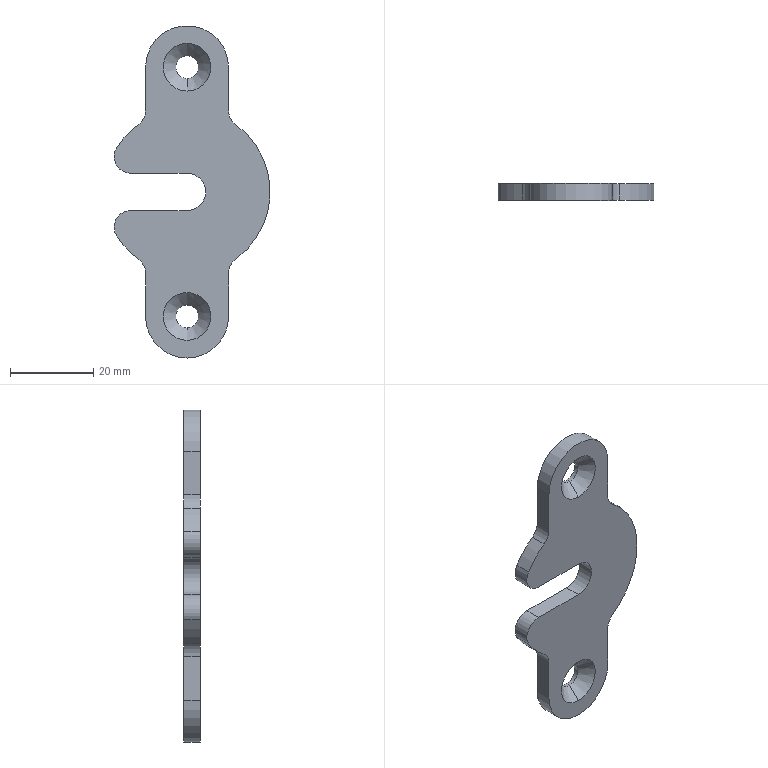Component | SolidWorks | QX1-16-BJPusherCylinderConnectionBlock-1 | 1 solid | 29 faces | box 37.56 x 4 x 80 mm | volume 6717 mm3 | cylinder 17 | plane 8 | cone 4 | commonest cylinder face diameters 8 x6 5.5 x4 20 x3 40 x3 9 x1 | material Q235
STEP:
#1=CARTESIAN_POINT('',(0.,-3.701,-1.289));
#2=VERTEX_POINT('',#1);
#3=CARTESIAN_POINT('',(0.,-3.701,-1.073));
#4=VERTEX_POINT('',#3);
#5=CARTESIAN_POINT('',(0.,-3.701,-1.181));
#6=DIRECTION('',(0.,-1.,0.));
#7=DIRECTION('',(0.,0.,-1.));
#8=AXIS2_PLACEMENT_3D('',#5,#6,#7);
#9=CIRCLE('',#8,0.1083);
#10=EDGE_CURVE('',#2,#4,#9,.T.);
#11=ORIENTED_EDGE('',*,*,#10,.F.);
#12=CARTESIAN_POINT('',(0.,-3.819,-1.407));
#13=VERTEX_POINT('',#12);
#14=CARTESIAN_POINT('',(0.,-3.701,-1.289));
#15=DIRECTION('',(0.,-0.7071,-0.7071));
#16=VECTOR('',#15,39.37);
#17=LINE('',#14,#16);
#18=EDGE_CURVE('',#2,#13,#17,.T.);
#19=ORIENTED_EDGE('',*,*,#18,.T.);
#20=CARTESIAN_POINT('',(0.,-3.819,-0.9547));
#21=VERTEX_POINT('',#20);
#22=CARTESIAN_POINT('',(0.,-3.819,-1.181));
#23=DIRECTION('',(-0.,1.,-0.));
#24=DIRECTION('',(0.,0.,-1.));
#25=AXIS2_PLACEMENT_3D('',#22,#23,#24);
#26=CIRCLE('',#25,0.2264);
#27=EDGE_CURVE('',#21,#13,#26,.T.);
#28=ORIENTED_EDGE('',*,*,#27,.F.);
#29=CARTESIAN_POINT('',(0.,-3.701,-1.073));
#30=DIRECTION('',(0.,-0.7071,0.7071));
#31=VECTOR('',#30,39.37);
#32=LINE('',#29,#31);
#33=EDGE_CURVE('',#4,#21,#32,.T.);
#34=ORIENTED_EDGE('',*,*,#33,.F.);
#35=EDGE_LOOP('',(#11,#19,#28,#34));
#36=FACE_OUTER_BOUND('',#35,.T.);
#37=CARTESIAN_POINT('',(0.,-3.701,-1.181));
#38=DIRECTION('',(0.,-1.,0.));
#39=DIRECTION('',(-0.,0.,1.));
#40=AXIS2_PLACEMENT_3D('',#37,#38,#39);
#41=CONICAL_SURFACE('',#40,0.1083,0.7854);
#42=ADVANCED_FACE('',(#36),#41,.F.);
#43=CARTESIAN_POINT('',(0.,-3.701,1.073));
#44=VERTEX_POINT('',#43);
#45=CARTESIAN_POINT('',(0.,-3.701,1.289));
#46=VERTEX_POINT('',#45);
#47=CARTESIAN_POINT('',(0.,-3.701,1.181));
#48=DIRECTION('',(0.,-1.,0.));
#49=DIRECTION('',(0.,0.,-1.));
#50=AXIS2_PLACEMENT_3D('',#47,#48,#49);
#51=CIRCLE('',#50,0.1083);
#52=EDGE_CURVE('',#44,#46,#51,.T.);
#53=ORIENTED_EDGE('',*,*,#52,.F.);
#54=CARTESIAN_POINT('',(0.,-3.819,0.9547));
#55=VERTEX_POINT('',#54);
#56=CARTESIAN_POINT('',(0.,-3.701,1.073));
#57=DIRECTION('',(0.,-0.7071,-0.7071));
#58=VECTOR('',#57,39.37);
#59=LINE('',#56,#58);
#60=EDGE_CURVE('',#44,#55,#59,.T.);
#61=ORIENTED_EDGE('',*,*,#60,.T.);
#62=CARTESIAN_POINT('',(0.,-3.819,1.407));
#63=VERTEX_POINT('',#62);
#64=CARTESIAN_POINT('',(0.,-3.819,1.181));
#65=DIRECTION('',(-0.,1.,-0.));
#66=DIRECTION('',(0.,0.,-1.));
#67=AXIS2_PLACEMENT_3D('',#64,#65,#66);
#68=CIRCLE('',#67,0.2264);
#69=EDGE_CURVE('',#63,#55,#68,.T.);
#70=ORIENTED_EDGE('',*,*,#69,.F.);
#71=CARTESIAN_POINT('',(0.,-3.701,1.289));
#72=DIRECTION('',(0.,-0.7071,0.7071));
#73=VECTOR('',#72,39.37);
#74=LINE('',#71,#73);
#75=EDGE_CURVE('',#46,#63,#74,.T.);
#76=ORIENTED_EDGE('',*,*,#75,.F.);
#77=EDGE_LOOP('',(#53,#61,#70,#76));
#78=FACE_OUTER_BOUND('',#77,.T.);
#79=CARTESIAN_POINT('',(0.,-3.701,1.181));
#80=DIRECTION('',(0.,-1.,0.));
#81=DIRECTION('',(-0.,0.,1.));
#82=AXIS2_PLACEMENT_3D('',#79,#80,#81);
#83=CONICAL_SURFACE('',#82,0.1083,0.7854);
#84=ADVANCED_FACE('',(#78),#83,.F.);
#85=CARTESIAN_POINT('',(0.,-3.661,-1.289));
#86=VERTEX_POINT('',#85);
#87=CARTESIAN_POINT('',(0.,-3.661,-1.073));
#88=VERTEX_POINT('',#87);
#89=CARTESIAN_POINT('',(0.,-3.661,-1.181));
#90=DIRECTION('',(0.,-1.,0.));
#91=DIRECTION('',(-0.,0.,1.));
#92=AXIS2_PLACEMENT_3D('',#89,#90,#91);
#93=CIRCLE('',#92,0.1083);
#94=EDGE_CURVE('',#86,#88,#93,.T.);
#95=ORIENTED_EDGE('',*,*,#94,.F.);
#96=CARTESIAN_POINT('',(0.,-3.819,-1.289));
#97=DIRECTION('',(0.,-1.,0.));
#98=VECTOR('',#97,39.37);
#99=LINE('',#96,#98);
#100=EDGE_CURVE('',#86,#2,#99,.T.);
#101=ORIENTED_EDGE('',*,*,#100,.T.);
#102=ORIENTED_EDGE('',*,*,#10,.T.);
#103=CARTESIAN_POINT('',(0.,-3.819,-1.073));
#104=DIRECTION('',(0.,-1.,0.));
#105=VECTOR('',#104,39.37);
#106=LINE('',#103,#105);
#107=EDGE_CURVE('',#88,#4,#106,.T.);
#108=ORIENTED_EDGE('',*,*,#107,.F.);
#109=EDGE_LOOP('',(#95,#101,#102,#108));
#110=FACE_OUTER_BOUND('',#109,.T.);
#111=CARTESIAN_POINT('',(0.,-3.819,-1.181));
#112=DIRECTION('',(0.,-1.,0.));
#113=DIRECTION('',(-0.,0.,1.));
#114=AXIS2_PLACEMENT_3D('',#111,#112,#113);
#115=CYLINDRICAL_SURFACE('',#114,0.1083);
#116=ADVANCED_FACE('',(#110),#115,.F.);
#117=CARTESIAN_POINT('',(0.,-3.661,1.073));
#118=VERTEX_POINT('',#117);
#119=CARTESIAN_POINT('',(0.,-3.661,1.289));
#120=VERTEX_POINT('',#119);
#121=CARTESIAN_POINT('',(0.,-3.661,1.181));
#122=DIRECTION('',(0.,-1.,0.));
#123=DIRECTION('',(-0.,0.,1.));
#124=AXIS2_PLACEMENT_3D('',#121,#122,#123);
#125=CIRCLE('',#124,0.1083);
#126=EDGE_CURVE('',#118,#120,#125,.T.);
#127=ORIENTED_EDGE('',*,*,#126,.F.);
#128=CARTESIAN_POINT('',(0.,-3.819,1.073));
#129=DIRECTION('',(0.,-1.,0.));
#130=VECTOR('',#129,39.37);
#131=LINE('',#128,#130);
#132=EDGE_CURVE('',#118,#44,#131,.T.);
#133=ORIENTED_EDGE('',*,*,#132,.T.);
#134=ORIENTED_EDGE('',*,*,#52,.T.);
#135=CARTESIAN_POINT('',(0.,-3.819,1.289));
#136=DIRECTION('',(0.,-1.,0.));
#137=VECTOR('',#136,39.37);
#138=LINE('',#135,#137);
#139=EDGE_CURVE('',#120,#46,#138,.T.);
#140=ORIENTED_EDGE('',*,*,#139,.F.);
#141=EDGE_LOOP('',(#127,#133,#134,#140));
#142=FACE_OUTER_BOUND('',#141,.T.);
#143=CARTESIAN_POINT('',(0.,-3.819,1.181));
#144=DIRECTION('',(0.,-1.,0.));
#145=DIRECTION('',(-0.,0.,1.));
#146=AXIS2_PLACEMENT_3D('',#143,#144,#145);
#147=CYLINDRICAL_SURFACE('',#146,0.1083);
#148=ADVANCED_FACE('',(#142),#147,.F.);
#149=CARTESIAN_POINT('',(0.3937,-3.819,-1.181));
#150=VERTEX_POINT('',#149);
#151=CARTESIAN_POINT('',(0.,-3.819,-1.575));
#152=VERTEX_POINT('',#151);
#153=CARTESIAN_POINT('',(0.,-3.819,-1.181));
#154=DIRECTION('',(-0.,1.,-0.));
#155=DIRECTION('',(0.,0.,-1.));
#156=AXIS2_PLACEMENT_3D('',#153,#154,#155);
#157=CIRCLE('',#156,0.3937);
#158=EDGE_CURVE('',#150,#152,#157,.T.);
#159=ORIENTED_EDGE('',*,*,#158,.T.);
#160=CARTESIAN_POINT('',(0.,-3.661,-1.575));
#161=VERTEX_POINT('',#160);
#162=CARTESIAN_POINT('',(0.,-3.819,-1.575));
#163=DIRECTION('',(-0.,1.,-0.));
#164=VECTOR('',#163,39.37);
#165=LINE('',#162,#164);
#166=EDGE_CURVE('',#152,#161,#165,.T.);
#167=ORIENTED_EDGE('',*,*,#166,.T.);
#168=CARTESIAN_POINT('',(0.3937,-3.661,-1.181));
#169=VERTEX_POINT('',#168);
#170=CARTESIAN_POINT('',(0.,-3.661,-1.181));
#171=DIRECTION('',(-0.,1.,-0.));
#172=DIRECTION('',(0.,0.,-1.));
#173=AXIS2_PLACEMENT_3D('',#170,#171,#172);
#174=CIRCLE('',#173,0.3937);
#175=EDGE_CURVE('',#169,#161,#174,.T.);
#176=ORIENTED_EDGE('',*,*,#175,.F.);
#177=CARTESIAN_POINT('',(0.3937,-3.819,-1.181));
#178=DIRECTION('',(-0.,1.,-0.));
#179=VECTOR('',#178,39.37);
#180=LINE('',#177,#179);
#181=EDGE_CURVE('',#150,#169,#180,.T.);
#182=ORIENTED_EDGE('',*,*,#181,.F.);
#183=EDGE_LOOP('',(#159,#167,#176,#182));
#184=FACE_OUTER_BOUND('',#183,.T.);
#185=CARTESIAN_POINT('',(0.,-3.819,-1.181));
#186=DIRECTION('',(-0.,1.,-0.));
#187=DIRECTION('',(0.,0.,-1.));
#188=AXIS2_PLACEMENT_3D('',#185,#186,#187);
#189=CYLINDRICAL_SURFACE('',#188,0.3937);
#190=ADVANCED_FACE('',(#184),#189,.T.);
#191=ORIENTED_EDGE('',*,*,#69,.T.);
#192=CARTESIAN_POINT('',(0.,-3.819,1.181));
#193=DIRECTION('',(-0.,1.,-0.));
#194=DIRECTION('',(0.,0.,-1.));
#195=AXIS2_PLACEMENT_3D('',#192,#193,#194);
#196=CIRCLE('',#195,0.2264);
#197=EDGE_CURVE('',#55,#63,#196,.T.);
#198=ORIENTED_EDGE('',*,*,#197,.T.);
#199=EDGE_LOOP('',(#191,#198));
#200=FACE_BOUND('',#199,.T.);
#201=ORIENTED_EDGE('',*,*,#27,.T.);
#202=CARTESIAN_POINT('',(0.,-3.819,-1.181));
#203=DIRECTION('',(-0.,1.,-0.));
#204=DIRECTION('',(0.,0.,-1.));
#205=AXIS2_PLACEMENT_3D('',#202,#203,#204);
#206=CIRCLE('',#205,0.2264);
#207=EDGE_CURVE('',#13,#21,#206,.T.);
#208=ORIENTED_EDGE('',*,*,#207,.T.);
#209=EDGE_LOOP('',(#201,#208));
#210=FACE_BOUND('',#209,.T.);
#211=CARTESIAN_POINT('',(0.,-3.819,-0.1772));
#212=VERTEX_POINT('',#211);
#213=CARTESIAN_POINT('',(-0.5337,-3.819,-0.1772));
#214=VERTEX_POINT('',#213);
#215=CARTESIAN_POINT('',(0.,-3.819,-0.1772));
#216=DIRECTION('',(-1.,-0.,-0.));
#217=VECTOR('',#216,39.37);
#218=LINE('',#215,#217);
#219=EDGE_CURVE('',#212,#214,#218,.T.);
#220=ORIENTED_EDGE('',*,*,#219,.T.);
#221=CARTESIAN_POINT('',(-0.6671,-3.819,-0.4183));
#222=VERTEX_POINT('',#221);
#223=CARTESIAN_POINT('',(-0.5337,-3.819,-0.3346));
#224=DIRECTION('',(0.,-1.,0.));
#225=DIRECTION('',(0.,0.,-1.));
#226=AXIS2_PLACEMENT_3D('',#223,#224,#225);
#227=CIRCLE('',#226,0.1575);
#228=EDGE_CURVE('',#214,#222,#227,.T.);
#229=ORIENTED_EDGE('',*,*,#228,.T.);
#230=CARTESIAN_POINT('',(-0.4593,-3.819,-0.6396));
#231=VERTEX_POINT('',#230);
#232=CARTESIAN_POINT('',(0.,-3.819,0.));
#233=DIRECTION('',(-0.,1.,-0.));
#234=DIRECTION('',(0.,0.,-1.));
#235=AXIS2_PLACEMENT_3D('',#232,#233,#234);
#236=CIRCLE('',#235,0.7874);
#237=EDGE_CURVE('',#231,#222,#236,.T.);
#238=ORIENTED_EDGE('',*,*,#237,.F.);
#239=CARTESIAN_POINT('',(-0.3937,-3.819,-0.7675));
#240=VERTEX_POINT('',#239);
#241=CARTESIAN_POINT('',(-0.5512,-3.819,-0.7675));
#242=DIRECTION('',(-0.,1.,-0.));
#243=DIRECTION('',(0.,0.,-1.));
#244=AXIS2_PLACEMENT_3D('',#241,#242,#243);
#245=CIRCLE('',#244,0.1575);
#246=EDGE_CURVE('',#231,#240,#245,.T.);
#247=ORIENTED_EDGE('',*,*,#246,.T.);
#248=CARTESIAN_POINT('',(-0.3937,-3.819,-1.181));
#249=VERTEX_POINT('',#248);
#250=CARTESIAN_POINT('',(-0.3937,-3.819,1.181));
#251=DIRECTION('',(-0.,0.,1.));
#252=VECTOR('',#251,39.37);
#253=LINE('',#250,#252);
#254=EDGE_CURVE('',#249,#240,#253,.T.);
#255=ORIENTED_EDGE('',*,*,#254,.F.);
#256=CARTESIAN_POINT('',(0.,-3.819,-1.181));
#257=DIRECTION('',(-0.,1.,-0.));
#258=DIRECTION('',(0.,0.,-1.));
#259=AXIS2_PLACEMENT_3D('',#256,#257,#258);
#260=CIRCLE('',#259,0.3937);
#261=EDGE_CURVE('',#152,#249,#260,.T.);
#262=ORIENTED_EDGE('',*,*,#261,.F.);
#263=ORIENTED_EDGE('',*,*,#158,.F.);
#264=CARTESIAN_POINT('',(0.3937,-3.819,-0.7675));
#265=VERTEX_POINT('',#264);
#266=CARTESIAN_POINT('',(0.3937,-3.819,1.181));
#267=DIRECTION('',(0.,-0.,-1.));
#268=VECTOR('',#267,39.37);
#269=LINE('',#266,#268);
#270=EDGE_CURVE('',#265,#150,#269,.T.);
#271=ORIENTED_EDGE('',*,*,#270,.F.);
#272=CARTESIAN_POINT('',(0.4593,-3.819,-0.6396));
#273=VERTEX_POINT('',#272);
#274=CARTESIAN_POINT('',(0.5512,-3.819,-0.7675));
#275=DIRECTION('',(-0.,1.,-0.));
#276=DIRECTION('',(0.,0.,-1.));
#277=AXIS2_PLACEMENT_3D('',#274,#275,#276);
#278=CIRCLE('',#277,0.1575);
#279=EDGE_CURVE('',#265,#273,#278,.T.);
#280=ORIENTED_EDGE('',*,*,#279,.T.);
#281=CARTESIAN_POINT('',(0.4593,-3.819,0.6396));
#282=VERTEX_POINT('',#281);
#283=CARTESIAN_POINT('',(0.,-3.819,0.));
#284=DIRECTION('',(-0.,1.,-0.));
#285=DIRECTION('',(0.,0.,-1.));
#286=AXIS2_PLACEMENT_3D('',#283,#284,#285);
#287=CIRCLE('',#286,0.7874);
#288=EDGE_CURVE('',#282,#273,#287,.T.);
#289=ORIENTED_EDGE('',*,*,#288,.F.);
#290=CARTESIAN_POINT('',(0.3937,-3.819,0.7675));
#291=VERTEX_POINT('',#290);
#292=CARTESIAN_POINT('',(0.5512,-3.819,0.7675));
#293=DIRECTION('',(-0.,1.,-0.));
#294=DIRECTION('',(0.,0.,-1.));
#295=AXIS2_PLACEMENT_3D('',#292,#293,#294);
#296=CIRCLE('',#295,0.1575);
#297=EDGE_CURVE('',#282,#291,#296,.T.);
#298=ORIENTED_EDGE('',*,*,#297,.T.);
#299=CARTESIAN_POINT('',(0.3937,-3.819,1.181));
#300=VERTEX_POINT('',#299);
#301=CARTESIAN_POINT('',(0.3937,-3.819,1.181));
#302=DIRECTION('',(0.,-0.,-1.));
#303=VECTOR('',#302,39.37);
#304=LINE('',#301,#303);
#305=EDGE_CURVE('',#300,#291,#304,.T.);
#306=ORIENTED_EDGE('',*,*,#305,.F.);
#307=CARTESIAN_POINT('',(-0.3937,-3.819,1.181));
#308=VERTEX_POINT('',#307);
#309=CARTESIAN_POINT('',(0.,-3.819,1.181));
#310=DIRECTION('',(-0.,1.,-0.));
#311=DIRECTION('',(0.,0.,-1.));
#312=AXIS2_PLACEMENT_3D('',#309,#310,#311);
#313=CIRCLE('',#312,0.3937);
#314=EDGE_CURVE('',#308,#300,#313,.T.);
#315=ORIENTED_EDGE('',*,*,#314,.F.);
#316=CARTESIAN_POINT('',(-0.3937,-3.819,0.7675));
#317=VERTEX_POINT('',#316);
#318=CARTESIAN_POINT('',(-0.3937,-3.819,1.181));
#319=DIRECTION('',(-0.,0.,1.));
#320=VECTOR('',#319,39.37);
#321=LINE('',#318,#320);
#322=EDGE_CURVE('',#317,#308,#321,.T.);
#323=ORIENTED_EDGE('',*,*,#322,.F.);
#324=CARTESIAN_POINT('',(-0.4593,-3.819,0.6396));
#325=VERTEX_POINT('',#324);
#326=CARTESIAN_POINT('',(-0.5512,-3.819,0.7675));
#327=DIRECTION('',(-0.,1.,-0.));
#328=DIRECTION('',(0.,0.,-1.));
#329=AXIS2_PLACEMENT_3D('',#326,#327,#328);
#330=CIRCLE('',#329,0.1575);
#331=EDGE_CURVE('',#317,#325,#330,.T.);
#332=ORIENTED_EDGE('',*,*,#331,.T.);
#333=CARTESIAN_POINT('',(-0.6671,-3.819,0.4183));
#334=VERTEX_POINT('',#333);
#335=CARTESIAN_POINT('',(0.,-3.819,0.));
#336=DIRECTION('',(-0.,1.,-0.));
#337=DIRECTION('',(0.,0.,-1.));
#338=AXIS2_PLACEMENT_3D('',#335,#336,#337);
#339=CIRCLE('',#338,0.7874);
#340=EDGE_CURVE('',#334,#325,#339,.T.);
#341=ORIENTED_EDGE('',*,*,#340,.F.);
#342=CARTESIAN_POINT('',(-0.5337,-3.819,0.1772));
#343=VERTEX_POINT('',#342);
#344=CARTESIAN_POINT('',(-0.5337,-3.819,0.3346));
#345=DIRECTION('',(0.,-1.,0.));
#346=DIRECTION('',(0.,0.,-1.));
#347=AXIS2_PLACEMENT_3D('',#344,#345,#346);
#348=CIRCLE('',#347,0.1575);
#349=EDGE_CURVE('',#334,#343,#348,.T.);
#350=ORIENTED_EDGE('',*,*,#349,.T.);
#351=CARTESIAN_POINT('',(0.,-3.819,0.1772));
#352=VERTEX_POINT('',#351);
#353=CARTESIAN_POINT('',(0.,-3.819,0.1772));
#354=DIRECTION('',(-1.,-0.,-0.));
#355=VECTOR('',#354,39.37);
#356=LINE('',#353,#355);
#357=EDGE_CURVE('',#352,#343,#356,.T.);
#358=ORIENTED_EDGE('',*,*,#357,.F.);
#359=CARTESIAN_POINT('',(0.,-3.819,0.));
#360=DIRECTION('',(-0.,1.,-0.));
#361=DIRECTION('',(0.,0.,-1.));
#362=AXIS2_PLACEMENT_3D('',#359,#360,#361);
#363=CIRCLE('',#362,0.1772);
#364=EDGE_CURVE('',#352,#212,#363,.T.);
#365=ORIENTED_EDGE('',*,*,#364,.T.);
#366=EDGE_LOOP('',(#220,#229,#238,#247,#255,#262,#263,#271,#280,#289,#298,#306,#315,#323,#332,#341,#350,#358,#365));
#367=FACE_OUTER_BOUND('',#366,.T.);
#368=CARTESIAN_POINT('',(0.,-3.819,1.181));
#369=DIRECTION('',(-0.,1.,-0.));
#370=DIRECTION('',(0.,-0.,-1.));
#371=AXIS2_PLACEMENT_3D('',#368,#369,#370);
#372=PLANE('',#371);
#373=ADVANCED_FACE('',(#200,#210,#367),#372,.F.);
#374=CARTESIAN_POINT('',(0.,-3.661,-1.181));
#375=DIRECTION('',(0.,-1.,0.));
#376=DIRECTION('',(-0.,0.,1.));
#377=AXIS2_PLACEMENT_3D('',#374,#375,#376);
#378=CIRCLE('',#377,0.1083);
#379=EDGE_CURVE('',#88,#86,#378,.T.);
#380=ORIENTED_EDGE('',*,*,#379,.T.);
#381=ORIENTED_EDGE('',*,*,#94,.T.);
#382=EDGE_LOOP('',(#380,#381));
#383=FACE_BOUND('',#382,.T.);
#384=CARTESIAN_POINT('',(-0.4593,-3.661,-0.6396));
#385=VERTEX_POINT('',#384);
#386=CARTESIAN_POINT('',(-0.6671,-3.661,-0.4183));
#387=VERTEX_POINT('',#386);
#388=CARTESIAN_POINT('',(0.,-3.661,0.));
#389=DIRECTION('',(-0.,1.,-0.));
#390=DIRECTION('',(0.,0.,-1.));
#391=AXIS2_PLACEMENT_3D('',#388,#389,#390);
#392=CIRCLE('',#391,0.7874);
#393=EDGE_CURVE('',#385,#387,#392,.T.);
#394=ORIENTED_EDGE('',*,*,#393,.T.);
#395=CARTESIAN_POINT('',(-0.5337,-3.661,-0.1772));
#396=VERTEX_POINT('',#395);
#397=CARTESIAN_POINT('',(-0.5337,-3.661,-0.3346));
#398=DIRECTION('',(-0.,1.,-0.));
#399=DIRECTION('',(0.,0.,-1.));
#400=AXIS2_PLACEMENT_3D('',#397,#398,#399);
#401=CIRCLE('',#400,0.1575);
#402=EDGE_CURVE('',#387,#396,#401,.T.);
#403=ORIENTED_EDGE('',*,*,#402,.T.);
#404=CARTESIAN_POINT('',(0.,-3.661,-0.1772));
#405=VERTEX_POINT('',#404);
#406=CARTESIAN_POINT('',(0.,-3.661,-0.1772));
#407=DIRECTION('',(-1.,-0.,-0.));
#408=VECTOR('',#407,39.37);
#409=LINE('',#406,#408);
#410=EDGE_CURVE('',#405,#396,#409,.T.);
#411=ORIENTED_EDGE('',*,*,#410,.F.);
#412=CARTESIAN_POINT('',(0.,-3.661,0.1772));
#413=VERTEX_POINT('',#412);
#414=CARTESIAN_POINT('',(0.,-3.661,0.));
#415=DIRECTION('',(-0.,1.,-0.));
#416=DIRECTION('',(0.,0.,-1.));
#417=AXIS2_PLACEMENT_3D('',#414,#415,#416);
#418=CIRCLE('',#417,0.1772);
#419=EDGE_CURVE('',#413,#405,#418,.T.);
#420=ORIENTED_EDGE('',*,*,#419,.F.);
#421=CARTESIAN_POINT('',(-0.5337,-3.661,0.1772));
#422=VERTEX_POINT('',#421);
#423=CARTESIAN_POINT('',(0.,-3.661,0.1772));
#424=DIRECTION('',(-1.,-0.,-0.));
#425=VECTOR('',#424,39.37);
#426=LINE('',#423,#425);
#427=EDGE_CURVE('',#413,#422,#426,.T.);
#428=ORIENTED_EDGE('',*,*,#427,.T.);
#429=CARTESIAN_POINT('',(-0.6671,-3.661,0.4183));
#430=VERTEX_POINT('',#429);
#431=CARTESIAN_POINT('',(-0.5337,-3.661,0.3346));
#432=DIRECTION('',(-0.,1.,-0.));
#433=DIRECTION('',(0.,0.,-1.));
#434=AXIS2_PLACEMENT_3D('',#431,#432,#433);
#435=CIRCLE('',#434,0.1575);
#436=EDGE_CURVE('',#422,#430,#435,.T.);
#437=ORIENTED_EDGE('',*,*,#436,.T.);
#438=CARTESIAN_POINT('',(-0.4593,-3.661,0.6396));
#439=VERTEX_POINT('',#438);
#440=CARTESIAN_POINT('',(0.,-3.661,0.));
#441=DIRECTION('',(-0.,1.,-0.));
#442=DIRECTION('',(0.,0.,-1.));
#443=AXIS2_PLACEMENT_3D('',#440,#441,#442);
#444=CIRCLE('',#443,0.7874);
#445=EDGE_CURVE('',#430,#439,#444,.T.);
#446=ORIENTED_EDGE('',*,*,#445,.T.);
#447=CARTESIAN_POINT('',(-0.3937,-3.661,0.7675));
#448=VERTEX_POINT('',#447);
#449=CARTESIAN_POINT('',(-0.5512,-3.661,0.7675));
#450=DIRECTION('',(0.,-1.,0.));
#451=DIRECTION('',(0.,0.,-1.));
#452=AXIS2_PLACEMENT_3D('',#449,#450,#451);
#453=CIRCLE('',#452,0.1575);
#454=EDGE_CURVE('',#439,#448,#453,.T.);
#455=ORIENTED_EDGE('',*,*,#454,.T.);
#456=CARTESIAN_POINT('',(-0.3937,-3.661,1.181));
#457=VERTEX_POINT('',#456);
#458=CARTESIAN_POINT('',(-0.3937,-3.661,1.181));
#459=DIRECTION('',(-0.,0.,1.));
#460=VECTOR('',#459,39.37);
#461=LINE('',#458,#460);
#462=EDGE_CURVE('',#448,#457,#461,.T.);
#463=ORIENTED_EDGE('',*,*,#462,.T.);
#464=CARTESIAN_POINT('',(0.3937,-3.661,1.181));
#465=VERTEX_POINT('',#464);
#466=CARTESIAN_POINT('',(0.,-3.661,1.181));
#467=DIRECTION('',(-0.,1.,-0.));
#468=DIRECTION('',(0.,0.,-1.));
#469=AXIS2_PLACEMENT_3D('',#466,#467,#468);
#470=CIRCLE('',#469,0.3937);
#471=EDGE_CURVE('',#457,#465,#470,.T.);
#472=ORIENTED_EDGE('',*,*,#471,.T.);
#473=CARTESIAN_POINT('',(0.3937,-3.661,0.7675));
#474=VERTEX_POINT('',#473);
#475=CARTESIAN_POINT('',(0.3937,-3.661,1.181));
#476=DIRECTION('',(0.,-0.,-1.));
#477=VECTOR('',#476,39.37);
#478=LINE('',#475,#477);
#479=EDGE_CURVE('',#465,#474,#478,.T.);
#480=ORIENTED_EDGE('',*,*,#479,.T.);
#481=CARTESIAN_POINT('',(0.4593,-3.661,0.6396));
#482=VERTEX_POINT('',#481);
#483=CARTESIAN_POINT('',(0.5512,-3.661,0.7675));
#484=DIRECTION('',(0.,-1.,0.));
#485=DIRECTION('',(-0.,0.,-1.));
#486=AXIS2_PLACEMENT_3D('',#483,#484,#485);
#487=CIRCLE('',#486,0.1575);
#488=EDGE_CURVE('',#474,#482,#487,.T.);
#489=ORIENTED_EDGE('',*,*,#488,.T.);
#490=CARTESIAN_POINT('',(0.4593,-3.661,-0.6396));
#491=VERTEX_POINT('',#490);
#492=CARTESIAN_POINT('',(0.,-3.661,0.));
#493=DIRECTION('',(-0.,1.,-0.));
#494=DIRECTION('',(0.,0.,-1.));
#495=AXIS2_PLACEMENT_3D('',#492,#493,#494);
#496=CIRCLE('',#495,0.7874);
#497=EDGE_CURVE('',#482,#491,#496,.T.);
#498=ORIENTED_EDGE('',*,*,#497,.T.);
#499=CARTESIAN_POINT('',(0.3937,-3.661,-0.7675));
#500=VERTEX_POINT('',#499);
#501=CARTESIAN_POINT('',(0.5512,-3.661,-0.7675));
#502=DIRECTION('',(0.,-1.,0.));
#503=DIRECTION('',(0.,0.,-1.));
#504=AXIS2_PLACEMENT_3D('',#501,#502,#503);
#505=CIRCLE('',#504,0.1575);
#506=EDGE_CURVE('',#491,#500,#505,.T.);
#507=ORIENTED_EDGE('',*,*,#506,.T.);
#508=CARTESIAN_POINT('',(0.3937,-3.661,1.181));
#509=DIRECTION('',(0.,-0.,-1.));
#510=VECTOR('',#509,39.37);
#511=LINE('',#508,#510);
#512=EDGE_CURVE('',#500,#169,#511,.T.);
#513=ORIENTED_EDGE('',*,*,#512,.T.);
#514=ORIENTED_EDGE('',*,*,#175,.T.);
#515=CARTESIAN_POINT('',(-0.3937,-3.661,-1.181));
#516=VERTEX_POINT('',#515);
#517=CARTESIAN_POINT('',(0.,-3.661,-1.181));
#518=DIRECTION('',(-0.,1.,-0.));
#519=DIRECTION('',(0.,0.,-1.));
#520=AXIS2_PLACEMENT_3D('',#517,#518,#519);
#521=CIRCLE('',#520,0.3937);
#522=EDGE_CURVE('',#161,#516,#521,.T.);
#523=ORIENTED_EDGE('',*,*,#522,.T.);
#524=CARTESIAN_POINT('',(-0.3937,-3.661,-0.7675));
#525=VERTEX_POINT('',#524);
#526=CARTESIAN_POINT('',(-0.3937,-3.661,1.181));
#527=DIRECTION('',(-0.,0.,1.));
#528=VECTOR('',#527,39.37);
#529=LINE('',#526,#528);
#530=EDGE_CURVE('',#516,#525,#529,.T.);
#531=ORIENTED_EDGE('',*,*,#530,.T.);
#532=CARTESIAN_POINT('',(-0.5512,-3.661,-0.7675));
#533=DIRECTION('',(0.,-1.,0.));
#534=DIRECTION('',(0.,0.,-1.));
#535=AXIS2_PLACEMENT_3D('',#532,#533,#534);
#536=CIRCLE('',#535,0.1575);
#537=EDGE_CURVE('',#525,#385,#536,.T.);
#538=ORIENTED_EDGE('',*,*,#537,.T.);
#539=EDGE_LOOP('',(#394,#403,#411,#420,#428,#437,#446,#455,#463,#472,#480,#489,#498,#507,#513,#514,#523,#531,#538));
#540=FACE_OUTER_BOUND('',#539,.T.);
#541=CARTESIAN_POINT('',(0.,-3.661,1.181));
#542=DIRECTION('',(0.,-1.,0.));
#543=DIRECTION('',(-0.,0.,1.));
#544=AXIS2_PLACEMENT_3D('',#541,#542,#543);
#545=CIRCLE('',#544,0.1083);
#546=EDGE_CURVE('',#120,#118,#545,.T.);
#547=ORIENTED_EDGE('',*,*,#546,.T.);
#548=ORIENTED_EDGE('',*,*,#126,.T.);
#549=EDGE_LOOP('',(#547,#548));
#550=FACE_BOUND('',#549,.T.);
#551=CARTESIAN_POINT('',(0.,-3.661,1.181));
#552=DIRECTION('',(-0.,1.,-0.));
#553=DIRECTION('',(0.,-0.,-1.));
#554=AXIS2_PLACEMENT_3D('',#551,#552,#553);
#555=PLANE('',#554);
#556=ADVANCED_FACE('',(#383,#540,#550),#555,.T.);
#557=ORIENTED_EDGE('',*,*,#512,.F.);
#558=CARTESIAN_POINT('',(0.3937,-3.819,-0.7675));
#559=DIRECTION('',(0.,-1.,0.));
#560=VECTOR('',#559,39.37);
#561=LINE('',#558,#560);
#562=EDGE_CURVE('',#500,#265,#561,.T.);
#563=ORIENTED_EDGE('',*,*,#562,.T.);
#564=ORIENTED_EDGE('',*,*,#270,.T.);
#565=ORIENTED_EDGE('',*,*,#181,.T.);
#566=EDGE_LOOP('',(#557,#563,#564,#565));
#567=FACE_OUTER_BOUND('',#566,.T.);
#568=CARTESIAN_POINT('',(0.3937,-3.819,1.181));
#569=DIRECTION('',(1.,0.,0.));
#570=DIRECTION('',(0.,-1.,0.));
#571=AXIS2_PLACEMENT_3D('',#568,#569,#570);
#572=PLANE('',#571);
#573=ADVANCED_FACE('',(#567),#572,.T.);
#574=ORIENTED_EDGE('',*,*,#462,.F.);
#575=CARTESIAN_POINT('',(-0.3937,-3.819,0.7675));
#576=DIRECTION('',(0.,-1.,0.));
#577=VECTOR('',#576,39.37);
#578=LINE('',#575,#577);
#579=EDGE_CURVE('',#448,#317,#578,.T.);
#580=ORIENTED_EDGE('',*,*,#579,.T.);
#581=ORIENTED_EDGE('',*,*,#322,.T.);
#582=CARTESIAN_POINT('',(-0.3937,-3.819,1.181));
#583=DIRECTION('',(-0.,1.,-0.));
#584=VECTOR('',#583,39.37);
#585=LINE('',#582,#584);
#586=EDGE_CURVE('',#308,#457,#585,.T.);
#587=ORIENTED_EDGE('',*,*,#586,.T.);
#588=EDGE_LOOP('',(#574,#580,#581,#587));
#589=FACE_OUTER_BOUND('',#588,.T.);
#590=CARTESIAN_POINT('',(-0.3937,-3.819,1.181));
#591=DIRECTION('',(-1.,-0.,-0.));
#592=DIRECTION('',(-0.,1.,-0.));
#593=AXIS2_PLACEMENT_3D('',#590,#591,#592);
#594=PLANE('',#593);
#595=ADVANCED_FACE('',(#589),#594,.T.);
#596=ORIENTED_EDGE('',*,*,#471,.F.);
#597=ORIENTED_EDGE('',*,*,#586,.F.);
#598=ORIENTED_EDGE('',*,*,#314,.T.);
#599=CARTESIAN_POINT('',(0.3937,-3.819,1.181));
#600=DIRECTION('',(-0.,1.,-0.));
#601=VECTOR('',#600,39.37);
#602=LINE('',#599,#601);
#603=EDGE_CURVE('',#300,#465,#602,.T.);
#604=ORIENTED_EDGE('',*,*,#603,.T.);
#605=EDGE_LOOP('',(#596,#597,#598,#604));
#606=FACE_OUTER_BOUND('',#605,.T.);
#607=CARTESIAN_POINT('',(0.,-3.819,1.181));
#608=DIRECTION('',(-0.,1.,-0.));
#609=DIRECTION('',(0.,0.,-1.));
#610=AXIS2_PLACEMENT_3D('',#607,#608,#609);
#611=CYLINDRICAL_SURFACE('',#610,0.3937);
#612=ADVANCED_FACE('',(#606),#611,.T.);
#613=ORIENTED_EDGE('',*,*,#254,.T.);
#614=CARTESIAN_POINT('',(-0.3937,-3.661,-0.7675));
#615=DIRECTION('',(-0.,1.,-0.));
#616=VECTOR('',#615,39.37);
#617=LINE('',#614,#616);
#618=EDGE_CURVE('',#240,#525,#617,.T.);
#619=ORIENTED_EDGE('',*,*,#618,.T.);
#620=ORIENTED_EDGE('',*,*,#530,.F.);
#621=CARTESIAN_POINT('',(-0.3937,-3.819,-1.181));
#622=DIRECTION('',(-0.,1.,-0.));
#623=VECTOR('',#622,39.37);
#624=LINE('',#621,#623);
#625=EDGE_CURVE('',#249,#516,#624,.T.);
#626=ORIENTED_EDGE('',*,*,#625,.F.);
#627=EDGE_LOOP('',(#613,#619,#620,#626));
#628=FACE_OUTER_BOUND('',#627,.T.);
#629=CARTESIAN_POINT('',(-0.3937,-3.819,1.181));
#630=DIRECTION('',(-1.,-0.,-0.));
#631=DIRECTION('',(-0.,1.,-0.));
#632=AXIS2_PLACEMENT_3D('',#629,#630,#631);
#633=PLANE('',#632);
#634=ADVANCED_FACE('',(#628),#633,.T.);
#635=ORIENTED_EDGE('',*,*,#166,.F.);
#636=ORIENTED_EDGE('',*,*,#261,.T.);
#637=ORIENTED_EDGE('',*,*,#625,.T.);
#638=ORIENTED_EDGE('',*,*,#522,.F.);
#639=EDGE_LOOP('',(#635,#636,#637,#638));
#640=FACE_OUTER_BOUND('',#639,.T.);
#641=CARTESIAN_POINT('',(0.,-3.819,-1.181));
#642=DIRECTION('',(-0.,1.,-0.));
#643=DIRECTION('',(0.,0.,-1.));
#644=AXIS2_PLACEMENT_3D('',#641,#642,#643);
#645=CYLINDRICAL_SURFACE('',#644,0.3937);
#646=ADVANCED_FACE('',(#640),#645,.T.);
#647=ORIENTED_EDGE('',*,*,#305,.T.);
#648=CARTESIAN_POINT('',(0.3937,-3.661,0.7675));
#649=DIRECTION('',(-0.,1.,-0.));
#650=VECTOR('',#649,39.37);
#651=LINE('',#648,#650);
#652=EDGE_CURVE('',#291,#474,#651,.T.);
#653=ORIENTED_EDGE('',*,*,#652,.T.);
#654=ORIENTED_EDGE('',*,*,#479,.F.);
#655=ORIENTED_EDGE('',*,*,#603,.F.);
#656=EDGE_LOOP('',(#647,#653,#654,#655));
#657=FACE_OUTER_BOUND('',#656,.T.);
#658=CARTESIAN_POINT('',(0.3937,-3.819,1.181));
#659=DIRECTION('',(1.,0.,0.));
#660=DIRECTION('',(0.,-1.,0.));
#661=AXIS2_PLACEMENT_3D('',#658,#659,#660);
#662=PLANE('',#661);
#663=ADVANCED_FACE('',(#657),#662,.T.);
#664=CARTESIAN_POINT('',(0.,-4.055,0.1772));
#665=DIRECTION('',(-0.,1.,-0.));
#666=VECTOR('',#665,39.37);
#667=LINE('',#664,#666);
#668=EDGE_CURVE('',#352,#413,#667,.T.);
#669=ORIENTED_EDGE('',*,*,#668,.T.);
#670=ORIENTED_EDGE('',*,*,#419,.T.);
#671=CARTESIAN_POINT('',(0.,-4.055,-0.1772));
#672=DIRECTION('',(-0.,1.,-0.));
#673=VECTOR('',#672,39.37);
#674=LINE('',#671,#673);
#675=EDGE_CURVE('',#212,#405,#674,.T.);
#676=ORIENTED_EDGE('',*,*,#675,.F.);
#677=ORIENTED_EDGE('',*,*,#364,.F.);
#678=EDGE_LOOP('',(#669,#670,#676,#677));
#679=FACE_OUTER_BOUND('',#678,.T.);
#680=CARTESIAN_POINT('',(0.,-4.055,0.));
#681=DIRECTION('',(-0.,1.,-0.));
#682=DIRECTION('',(0.,0.,-1.));
#683=AXIS2_PLACEMENT_3D('',#680,#681,#682);
#684=CYLINDRICAL_SURFACE('',#683,0.1772);
#685=ADVANCED_FACE('',(#679),#684,.F.);
#686=ORIENTED_EDGE('',*,*,#357,.T.);
#687=CARTESIAN_POINT('',(-0.5337,-4.055,0.1772));
#688=DIRECTION('',(-0.,1.,-0.));
#689=VECTOR('',#688,39.37);
#690=LINE('',#687,#689);
#691=EDGE_CURVE('',#343,#422,#690,.T.);
#692=ORIENTED_EDGE('',*,*,#691,.T.);
#693=ORIENTED_EDGE('',*,*,#427,.F.);
#694=ORIENTED_EDGE('',*,*,#668,.F.);
#695=EDGE_LOOP('',(#686,#692,#693,#694));
#696=FACE_OUTER_BOUND('',#695,.T.);
#697=CARTESIAN_POINT('',(0.,-4.055,0.1772));
#698=DIRECTION('',(0.,-0.,-1.));
#699=DIRECTION('',(0.,-1.,0.));
#700=AXIS2_PLACEMENT_3D('',#697,#698,#699);
#701=PLANE('',#700);
#702=ADVANCED_FACE('',(#696),#701,.T.);
#703=ORIENTED_EDGE('',*,*,#410,.T.);
#704=CARTESIAN_POINT('',(-0.5337,-3.819,-0.1772));
#705=DIRECTION('',(0.,-1.,0.));
#706=VECTOR('',#705,39.37);
#707=LINE('',#704,#706);
#708=EDGE_CURVE('',#396,#214,#707,.T.);
#709=ORIENTED_EDGE('',*,*,#708,.T.);
#710=ORIENTED_EDGE('',*,*,#219,.F.);
#711=ORIENTED_EDGE('',*,*,#675,.T.);
#712=EDGE_LOOP('',(#703,#709,#710,#711));
#713=FACE_OUTER_BOUND('',#712,.T.);
#714=CARTESIAN_POINT('',(0.,-4.055,-0.1772));
#715=DIRECTION('',(0.,-0.,-1.));
#716=DIRECTION('',(0.,-1.,0.));
#717=AXIS2_PLACEMENT_3D('',#714,#715,#716);
#718=PLANE('',#717);
#719=ADVANCED_FACE('',(#713),#718,.F.);
#720=ORIENTED_EDGE('',*,*,#340,.T.);
#721=CARTESIAN_POINT('',(-0.4593,-3.819,0.6396));
#722=DIRECTION('',(-0.,1.,-0.));
#723=VECTOR('',#722,39.37);
#724=LINE('',#721,#723);
#725=EDGE_CURVE('',#325,#439,#724,.T.);
#726=ORIENTED_EDGE('',*,*,#725,.T.);
#727=ORIENTED_EDGE('',*,*,#445,.F.);
#728=CARTESIAN_POINT('',(-0.6671,-3.819,0.4183));
#729=DIRECTION('',(0.,-1.,0.));
#730=VECTOR('',#729,39.37);
#731=LINE('',#728,#730);
#732=EDGE_CURVE('',#430,#334,#731,.T.);
#733=ORIENTED_EDGE('',*,*,#732,.T.);
#734=EDGE_LOOP('',(#720,#726,#727,#733));
#735=FACE_OUTER_BOUND('',#734,.T.);
#736=CARTESIAN_POINT('',(0.,-3.819,0.));
#737=DIRECTION('',(-0.,1.,-0.));
#738=DIRECTION('',(0.,0.,-1.));
#739=AXIS2_PLACEMENT_3D('',#736,#737,#738);
#740=CYLINDRICAL_SURFACE('',#739,0.7874);
#741=ADVANCED_FACE('',(#735),#740,.T.);
#742=ORIENTED_EDGE('',*,*,#393,.F.);
#743=CARTESIAN_POINT('',(-0.4593,-3.819,-0.6396));
#744=DIRECTION('',(0.,-1.,0.));
#745=VECTOR('',#744,39.37);
#746=LINE('',#743,#745);
#747=EDGE_CURVE('',#385,#231,#746,.T.);
#748=ORIENTED_EDGE('',*,*,#747,.T.);
#749=ORIENTED_EDGE('',*,*,#237,.T.);
#750=CARTESIAN_POINT('',(-0.6671,-3.819,-0.4183));
#751=DIRECTION('',(-0.,1.,-0.));
#752=VECTOR('',#751,39.37);
#753=LINE('',#750,#752);
#754=EDGE_CURVE('',#222,#387,#753,.T.);
#755=ORIENTED_EDGE('',*,*,#754,.T.);
#756=EDGE_LOOP('',(#742,#748,#749,#755));
#757=FACE_OUTER_BOUND('',#756,.T.);
#758=CARTESIAN_POINT('',(0.,-3.819,0.));
#759=DIRECTION('',(-0.,1.,-0.));
#760=DIRECTION('',(0.,0.,-1.));
#761=AXIS2_PLACEMENT_3D('',#758,#759,#760);
#762=CYLINDRICAL_SURFACE('',#761,0.7874);
#763=ADVANCED_FACE('',(#757),#762,.T.);
#764=ORIENTED_EDGE('',*,*,#497,.F.);
#765=CARTESIAN_POINT('',(0.4593,-3.819,0.6396));
#766=DIRECTION('',(0.,-1.,0.));
#767=VECTOR('',#766,39.37);
#768=LINE('',#765,#767);
#769=EDGE_CURVE('',#482,#282,#768,.T.);
#770=ORIENTED_EDGE('',*,*,#769,.T.);
#771=ORIENTED_EDGE('',*,*,#288,.T.);
#772=CARTESIAN_POINT('',(0.4593,-3.819,-0.6396));
#773=DIRECTION('',(-0.,1.,-0.));
#774=VECTOR('',#773,39.37);
#775=LINE('',#772,#774);
#776=EDGE_CURVE('',#273,#491,#775,.T.);
#777=ORIENTED_EDGE('',*,*,#776,.T.);
#778=EDGE_LOOP('',(#764,#770,#771,#777));
#779=FACE_OUTER_BOUND('',#778,.T.);
#780=CARTESIAN_POINT('',(0.,-3.819,0.));
#781=DIRECTION('',(-0.,1.,-0.));
#782=DIRECTION('',(0.,0.,-1.));
#783=AXIS2_PLACEMENT_3D('',#780,#781,#782);
#784=CYLINDRICAL_SURFACE('',#783,0.7874);
#785=ADVANCED_FACE('',(#779),#784,.T.);
#786=ORIENTED_EDGE('',*,*,#246,.F.);
#787=ORIENTED_EDGE('',*,*,#747,.F.);
#788=ORIENTED_EDGE('',*,*,#537,.F.);
#789=ORIENTED_EDGE('',*,*,#618,.F.);
#790=EDGE_LOOP('',(#786,#787,#788,#789));
#791=FACE_OUTER_BOUND('',#790,.T.);
#792=CARTESIAN_POINT('',(-0.5512,-3.819,-0.7675));
#793=DIRECTION('',(-0.,1.,-0.));
#794=DIRECTION('',(0.,0.,-1.));
#795=AXIS2_PLACEMENT_3D('',#792,#793,#794);
#796=CYLINDRICAL_SURFACE('',#795,0.1575);
#797=ADVANCED_FACE('',(#791),#796,.F.);
#798=ORIENTED_EDGE('',*,*,#331,.F.);
#799=ORIENTED_EDGE('',*,*,#579,.F.);
#800=ORIENTED_EDGE('',*,*,#454,.F.);
#801=ORIENTED_EDGE('',*,*,#725,.F.);
#802=EDGE_LOOP('',(#798,#799,#800,#801));
#803=FACE_OUTER_BOUND('',#802,.T.);
#804=CARTESIAN_POINT('',(-0.5512,-3.819,0.7675));
#805=DIRECTION('',(-0.,1.,-0.));
#806=DIRECTION('',(0.,0.,-1.));
#807=AXIS2_PLACEMENT_3D('',#804,#805,#806);
#808=CYLINDRICAL_SURFACE('',#807,0.1575);
#809=ADVANCED_FACE('',(#803),#808,.F.);
#810=ORIENTED_EDGE('',*,*,#297,.F.);
#811=ORIENTED_EDGE('',*,*,#769,.F.);
#812=ORIENTED_EDGE('',*,*,#488,.F.);
#813=ORIENTED_EDGE('',*,*,#652,.F.);
#814=EDGE_LOOP('',(#810,#811,#812,#813));
#815=FACE_OUTER_BOUND('',#814,.T.);
#816=CARTESIAN_POINT('',(0.5512,-3.819,0.7675));
#817=DIRECTION('',(-0.,1.,-0.));
#818=DIRECTION('',(0.,0.,-1.));
#819=AXIS2_PLACEMENT_3D('',#816,#817,#818);
#820=CYLINDRICAL_SURFACE('',#819,0.1575);
#821=ADVANCED_FACE('',(#815),#820,.F.);
#822=ORIENTED_EDGE('',*,*,#279,.F.);
#823=ORIENTED_EDGE('',*,*,#562,.F.);
#824=ORIENTED_EDGE('',*,*,#506,.F.);
#825=ORIENTED_EDGE('',*,*,#776,.F.);
#826=EDGE_LOOP('',(#822,#823,#824,#825));
#827=FACE_OUTER_BOUND('',#826,.T.);
#828=CARTESIAN_POINT('',(0.5512,-3.819,-0.7675));
#829=DIRECTION('',(-0.,1.,-0.));
#830=DIRECTION('',(0.,0.,-1.));
#831=AXIS2_PLACEMENT_3D('',#828,#829,#830);
#832=CYLINDRICAL_SURFACE('',#831,0.1575);
#833=ADVANCED_FACE('',(#827),#832,.F.);
#834=ORIENTED_EDGE('',*,*,#228,.F.);
#835=ORIENTED_EDGE('',*,*,#708,.F.);
#836=ORIENTED_EDGE('',*,*,#402,.F.);
#837=ORIENTED_EDGE('',*,*,#754,.F.);
#838=EDGE_LOOP('',(#834,#835,#836,#837));
#839=FACE_OUTER_BOUND('',#838,.T.);
#840=CARTESIAN_POINT('',(-0.5337,-3.819,-0.3346));
#841=DIRECTION('',(-0.,1.,-0.));
#842=DIRECTION('',(0.,0.,-1.));
#843=AXIS2_PLACEMENT_3D('',#840,#841,#842);
#844=CYLINDRICAL_SURFACE('',#843,0.1575);
#845=ADVANCED_FACE('',(#839),#844,.T.);
#846=ORIENTED_EDGE('',*,*,#349,.F.);
#847=ORIENTED_EDGE('',*,*,#732,.F.);
#848=ORIENTED_EDGE('',*,*,#436,.F.);
#849=ORIENTED_EDGE('',*,*,#691,.F.);
#850=EDGE_LOOP('',(#846,#847,#848,#849));
#851=FACE_OUTER_BOUND('',#850,.T.);
#852=CARTESIAN_POINT('',(-0.5337,-3.819,0.3346));
#853=DIRECTION('',(-0.,1.,-0.));
#854=DIRECTION('',(0.,0.,-1.));
#855=AXIS2_PLACEMENT_3D('',#852,#853,#854);
#856=CYLINDRICAL_SURFACE('',#855,0.1575);
#857=ADVANCED_FACE('',(#851),#856,.T.);
#858=ORIENTED_EDGE('',*,*,#132,.F.);
#859=ORIENTED_EDGE('',*,*,#546,.F.);
#860=ORIENTED_EDGE('',*,*,#139,.T.);
#861=CARTESIAN_POINT('',(0.,-3.701,1.181));
#862=DIRECTION('',(0.,-1.,0.));
#863=DIRECTION('',(0.,0.,-1.));
#864=AXIS2_PLACEMENT_3D('',#861,#862,#863);
#865=CIRCLE('',#864,0.1083);
#866=EDGE_CURVE('',#46,#44,#865,.T.);
#867=ORIENTED_EDGE('',*,*,#866,.T.);
#868=EDGE_LOOP('',(#858,#859,#860,#867));
#869=FACE_OUTER_BOUND('',#868,.T.);
#870=CARTESIAN_POINT('',(0.,-3.819,1.181));
#871=DIRECTION('',(0.,-1.,0.));
#872=DIRECTION('',(-0.,0.,1.));
#873=AXIS2_PLACEMENT_3D('',#870,#871,#872);
#874=CYLINDRICAL_SURFACE('',#873,0.1083);
#875=ADVANCED_FACE('',(#869),#874,.F.);
#876=ORIENTED_EDGE('',*,*,#100,.F.);
#877=ORIENTED_EDGE('',*,*,#379,.F.);
#878=ORIENTED_EDGE('',*,*,#107,.T.);
#879=CARTESIAN_POINT('',(0.,-3.701,-1.181));
#880=DIRECTION('',(0.,-1.,0.));
#881=DIRECTION('',(0.,0.,-1.));
#882=AXIS2_PLACEMENT_3D('',#879,#880,#881);
#883=CIRCLE('',#882,0.1083);
#884=EDGE_CURVE('',#4,#2,#883,.T.);
#885=ORIENTED_EDGE('',*,*,#884,.T.);
#886=EDGE_LOOP('',(#876,#877,#878,#885));
#887=FACE_OUTER_BOUND('',#886,.T.);
#888=CARTESIAN_POINT('',(0.,-3.819,-1.181));
#889=DIRECTION('',(0.,-1.,0.));
#890=DIRECTION('',(-0.,0.,1.));
#891=AXIS2_PLACEMENT_3D('',#888,#889,#890);
#892=CYLINDRICAL_SURFACE('',#891,0.1083);
#893=ADVANCED_FACE('',(#887),#892,.F.);
#894=ORIENTED_EDGE('',*,*,#60,.F.);
#895=ORIENTED_EDGE('',*,*,#866,.F.);
#896=ORIENTED_EDGE('',*,*,#75,.T.);
#897=ORIENTED_EDGE('',*,*,#197,.F.);
#898=EDGE_LOOP('',(#894,#895,#896,#897));
#899=FACE_OUTER_BOUND('',#898,.T.);
#900=CARTESIAN_POINT('',(0.,-3.701,1.181));
#901=DIRECTION('',(0.,-1.,0.));
#902=DIRECTION('',(-0.,0.,1.));
#903=AXIS2_PLACEMENT_3D('',#900,#901,#902);
#904=CONICAL_SURFACE('',#903,0.1083,0.7854);
#905=ADVANCED_FACE('',(#899),#904,.F.);
#906=ORIENTED_EDGE('',*,*,#18,.F.);
#907=ORIENTED_EDGE('',*,*,#884,.F.);
#908=ORIENTED_EDGE('',*,*,#33,.T.);
#909=ORIENTED_EDGE('',*,*,#207,.F.);
#910=EDGE_LOOP('',(#906,#907,#908,#909));
#911=FACE_OUTER_BOUND('',#910,.T.);
#912=CARTESIAN_POINT('',(0.,-3.701,-1.181));
#913=DIRECTION('',(0.,-1.,0.));
#914=DIRECTION('',(-0.,0.,1.));
#915=AXIS2_PLACEMENT_3D('',#912,#913,#914);
#916=CONICAL_SURFACE('',#915,0.1083,0.7854);
#917=ADVANCED_FACE('',(#911),#916,.F.);
#918=CLOSED_SHELL('',(#42,#84,#116,#148,#190,#373,#556,#573,#595,#612,#634,#646,#663,#685,#702,#719,#741,#763,#785,#797,#809,#821,#833,#845,#857,#875,#893,#905,#917));
#919=MANIFOLD_SOLID_BREP('',#918);
#920=CARTESIAN_POINT('',(0.,0.,0.));
#921=DIRECTION('',(0.,0.,1.));
#922=DIRECTION('',(1.,0.,0.));
#923=AXIS2_PLACEMENT_3D('',#920,#921,#922);
#924=(LENGTH_UNIT()NAMED_UNIT(*)SI_UNIT($,.METRE.));
#925=LENGTH_MEASURE_WITH_UNIT(LENGTH_MEASURE(0.0254),#924);
#926=DIMENSIONAL_EXPONENTS(1.,0.,0.,0.,0.,0.,0.);
#927=(CONVERSION_BASED_UNIT('',#925)LENGTH_UNIT()NAMED_UNIT(#926));
#928=UNCERTAINTY_MEASURE_WITH_UNIT(LENGTH_MEASURE(0.00001),#927,'','');
#929=(NAMED_UNIT(*)PLANE_ANGLE_UNIT()SI_UNIT($,.RADIAN.));
#930=(NAMED_UNIT(*)SI_UNIT($,.STERADIAN.)SOLID_ANGLE_UNIT());
#931=(GEOMETRIC_REPRESENTATION_CONTEXT(3)GLOBAL_UNCERTAINTY_ASSIGNED_CONTEXT((#928))GLOBAL_UNIT_ASSIGNED_CONTEXT((#927,#929,#930))REPRESENTATION_CONTEXT('',''));
#932=ADVANCED_BREP_SHAPE_REPRESENTATION('',(#919,#923),#931);
#933=COLOUR_RGB('',0.7922,0.8196,0.9333);
#934=FILL_AREA_STYLE_COLOUR('',#933);
#935=FILL_AREA_STYLE('',(#934));
#936=SURFACE_STYLE_FILL_AREA(#935);
#937=SURFACE_SIDE_STYLE('',(#936));
#938=SURFACE_STYLE_USAGE(.BOTH.,#937);
#939=PRESENTATION_STYLE_ASSIGNMENT((#938));
#940=STYLED_ITEM('',(#939),#919);
#941=(LENGTH_UNIT()NAMED_UNIT(*)SI_UNIT($,.METRE.));
#942=LENGTH_MEASURE_WITH_UNIT(LENGTH_MEASURE(0.0254),#941);
#943=DIMENSIONAL_EXPONENTS(1.,0.,0.,0.,0.,0.,0.);
#944=(CONVERSION_BASED_UNIT('',#942)LENGTH_UNIT()NAMED_UNIT(#943));
#945=UNCERTAINTY_MEASURE_WITH_UNIT(LENGTH_MEASURE(0.00001),#944,'','');
#946=(NAMED_UNIT(*)PLANE_ANGLE_UNIT()SI_UNIT($,.RADIAN.));
#947=(NAMED_UNIT(*)SI_UNIT($,.STERADIAN.)SOLID_ANGLE_UNIT());
#948=(GEOMETRIC_REPRESENTATION_CONTEXT(3)GLOBAL_UNCERTAINTY_ASSIGNED_CONTEXT((#945))GLOBAL_UNIT_ASSIGNED_CONTEXT((#944,#946,#947))REPRESENTATION_CONTEXT('',''));
#949=MECHANICAL_DESIGN_GEOMETRIC_PRESENTATION_REPRESENTATION('',(#940),#948);
#950=PRESENTATION_LAYER_ASSIGNMENT('','',(#940));